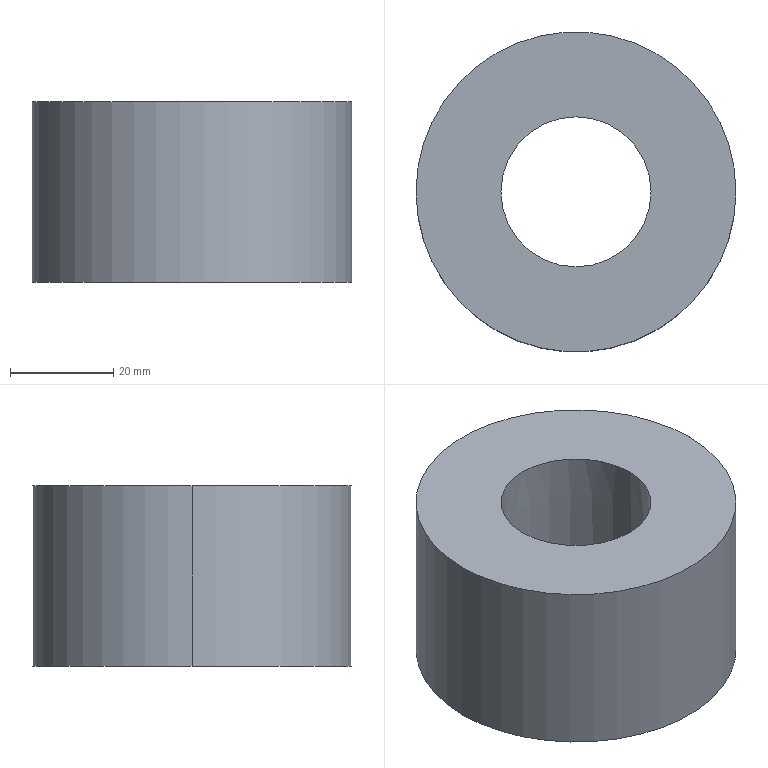Component | SolidWorks | JF21-80.1-1-3(_)-1-SOLID15-1 | 1 solid | 6 faces | box 62 x 62 x 35 mm | volume 80600 mm3 | cone 2 | cylinder 2 | plane 2 | commonest cylinder face diameters 62 x2
STEP:
#1=COLOUR_RGB('',0.7922,0.8196,0.9333);
#2=FILL_AREA_STYLE_COLOUR('',#1);
#3=FILL_AREA_STYLE('',(#2));
#4=SURFACE_STYLE_FILL_AREA(#3);
#5=SURFACE_SIDE_STYLE('',(#4));
#6=SURFACE_STYLE_USAGE(.BOTH.,#5);
#7=PRESENTATION_STYLE_ASSIGNMENT((#6));
#8=CARTESIAN_POINT('',(0.5728,-39.37,30.709));
#9=VERTEX_POINT('',#8);
#10=CARTESIAN_POINT('',(-0.5728,-39.37,30.709));
#11=VERTEX_POINT('',#10);
#12=CARTESIAN_POINT('',(0.,-39.37,30.709));
#13=DIRECTION('',(0.,0.,-1.));
#14=DIRECTION('',(-1.,0.,0.));
#15=AXIS2_PLACEMENT_3D('',#12,#13,#14);
#16=CIRCLE('',#15,0.5728);
#17=EDGE_CURVE('',#9,#11,#16,.T.);
#18=ORIENTED_EDGE('',*,*,#17,.F.);
#19=CARTESIAN_POINT('',(0.6158,-39.37,29.331));
#20=VERTEX_POINT('',#19);
#21=CARTESIAN_POINT('',(0.6158,-39.37,29.331));
#22=DIRECTION('',(-0.0312,-0.,0.9995));
#23=VECTOR('',#22,39.37);
#24=LINE('',#21,#23);
#25=EDGE_CURVE('',#20,#9,#24,.T.);
#26=ORIENTED_EDGE('',*,*,#25,.F.);
#27=CARTESIAN_POINT('',(-0.6158,-39.37,29.331));
#28=VERTEX_POINT('',#27);
#29=CARTESIAN_POINT('',(0.,-39.37,29.331));
#30=DIRECTION('',(0.,0.,-1.));
#31=DIRECTION('',(-1.,0.,0.));
#32=AXIS2_PLACEMENT_3D('',#29,#30,#31);
#33=CIRCLE('',#32,0.6158);
#34=EDGE_CURVE('',#20,#28,#33,.T.);
#35=ORIENTED_EDGE('',*,*,#34,.T.);
#36=CARTESIAN_POINT('',(-0.6158,-39.37,29.331));
#37=DIRECTION('',(0.0312,0.,0.9995));
#38=VECTOR('',#37,39.37);
#39=LINE('',#36,#38);
#40=EDGE_CURVE('',#28,#11,#39,.T.);
#41=ORIENTED_EDGE('',*,*,#40,.T.);
#42=EDGE_LOOP('',(#18,#26,#35,#41));
#43=FACE_OUTER_BOUND('',#42,.T.);
#44=CARTESIAN_POINT('',(0.,-39.37,29.331));
#45=DIRECTION('',(0.,0.,-1.));
#46=DIRECTION('',(1.,0.,0.));
#47=AXIS2_PLACEMENT_3D('',#44,#45,#46);
#48=CONICAL_SURFACE('',#47,0.6158,0.03121);
#49=ADVANCED_FACE('',(#43),#48,.F.);
#50=CARTESIAN_POINT('',(1.22,-39.37,30.709));
#51=VERTEX_POINT('',#50);
#52=CARTESIAN_POINT('',(-1.22,-39.37,30.709));
#53=VERTEX_POINT('',#52);
#54=CARTESIAN_POINT('',(0.,-39.37,30.709));
#55=DIRECTION('',(0.,0.,1.));
#56=DIRECTION('',(1.,0.,0.));
#57=AXIS2_PLACEMENT_3D('',#54,#55,#56);
#58=CIRCLE('',#57,1.22);
#59=EDGE_CURVE('',#51,#53,#58,.T.);
#60=ORIENTED_EDGE('',*,*,#59,.F.);
#61=CARTESIAN_POINT('',(1.22,-39.37,29.331));
#62=VERTEX_POINT('',#61);
#63=CARTESIAN_POINT('',(1.22,-39.37,30.709));
#64=DIRECTION('',(0.,0.,1.));
#65=VECTOR('',#64,39.37);
#66=LINE('',#63,#65);
#67=EDGE_CURVE('',#62,#51,#66,.T.);
#68=ORIENTED_EDGE('',*,*,#67,.F.);
#69=CARTESIAN_POINT('',(-1.22,-39.37,29.331));
#70=VERTEX_POINT('',#69);
#71=CARTESIAN_POINT('',(0.,-39.37,29.331));
#72=DIRECTION('',(0.,0.,1.));
#73=DIRECTION('',(1.,0.,0.));
#74=AXIS2_PLACEMENT_3D('',#71,#72,#73);
#75=CIRCLE('',#74,1.22);
#76=EDGE_CURVE('',#62,#70,#75,.T.);
#77=ORIENTED_EDGE('',*,*,#76,.T.);
#78=CARTESIAN_POINT('',(-1.22,-39.37,30.709));
#79=DIRECTION('',(0.,0.,1.));
#80=VECTOR('',#79,39.37);
#81=LINE('',#78,#80);
#82=EDGE_CURVE('',#70,#53,#81,.T.);
#83=ORIENTED_EDGE('',*,*,#82,.T.);
#84=EDGE_LOOP('',(#60,#68,#77,#83));
#85=FACE_OUTER_BOUND('',#84,.T.);
#86=CARTESIAN_POINT('',(0.,-39.37,30.709));
#87=DIRECTION('',(0.,0.,-1.));
#88=DIRECTION('',(1.,0.,0.));
#89=AXIS2_PLACEMENT_3D('',#86,#87,#88);
#90=CYLINDRICAL_SURFACE('',#89,1.22);
#91=ADVANCED_FACE('',(#85),#90,.T.);
#92=ORIENTED_EDGE('',*,*,#67,.T.);
#93=CARTESIAN_POINT('',(0.,-39.37,30.709));
#94=DIRECTION('',(0.,0.,1.));
#95=DIRECTION('',(1.,0.,0.));
#96=AXIS2_PLACEMENT_3D('',#93,#94,#95);
#97=CIRCLE('',#96,1.22);
#98=EDGE_CURVE('',#53,#51,#97,.T.);
#99=ORIENTED_EDGE('',*,*,#98,.F.);
#100=ORIENTED_EDGE('',*,*,#82,.F.);
#101=CARTESIAN_POINT('',(0.,-39.37,29.331));
#102=DIRECTION('',(0.,0.,1.));
#103=DIRECTION('',(1.,0.,0.));
#104=AXIS2_PLACEMENT_3D('',#101,#102,#103);
#105=CIRCLE('',#104,1.22);
#106=EDGE_CURVE('',#70,#62,#105,.T.);
#107=ORIENTED_EDGE('',*,*,#106,.T.);
#108=EDGE_LOOP('',(#92,#99,#100,#107));
#109=FACE_OUTER_BOUND('',#108,.T.);
#110=CARTESIAN_POINT('',(0.,-39.37,30.709));
#111=DIRECTION('',(0.,0.,-1.));
#112=DIRECTION('',(1.,0.,0.));
#113=AXIS2_PLACEMENT_3D('',#110,#111,#112);
#114=CYLINDRICAL_SURFACE('',#113,1.22);
#115=ADVANCED_FACE('',(#109),#114,.T.);
#116=CARTESIAN_POINT('',(0.,-39.37,30.709));
#117=DIRECTION('',(0.,0.,-1.));
#118=DIRECTION('',(-1.,0.,0.));
#119=AXIS2_PLACEMENT_3D('',#116,#117,#118);
#120=CIRCLE('',#119,0.5728);
#121=EDGE_CURVE('',#11,#9,#120,.T.);
#122=ORIENTED_EDGE('',*,*,#121,.T.);
#123=ORIENTED_EDGE('',*,*,#17,.T.);
#124=EDGE_LOOP('',(#122,#123));
#125=FACE_BOUND('',#124,.T.);
#126=ORIENTED_EDGE('',*,*,#98,.T.);
#127=ORIENTED_EDGE('',*,*,#59,.T.);
#128=EDGE_LOOP('',(#126,#127));
#129=FACE_OUTER_BOUND('',#128,.T.);
#130=CARTESIAN_POINT('',(0.,-39.37,30.709));
#131=DIRECTION('',(0.,0.,1.));
#132=DIRECTION('',(-1.,0.,0.));
#133=AXIS2_PLACEMENT_3D('',#130,#131,#132);
#134=PLANE('',#133);
#135=ADVANCED_FACE('',(#125,#129),#134,.T.);
#136=CARTESIAN_POINT('',(0.,-39.37,29.331));
#137=DIRECTION('',(0.,0.,-1.));
#138=DIRECTION('',(-1.,0.,0.));
#139=AXIS2_PLACEMENT_3D('',#136,#137,#138);
#140=CIRCLE('',#139,0.6158);
#141=EDGE_CURVE('',#28,#20,#140,.T.);
#142=ORIENTED_EDGE('',*,*,#141,.F.);
#143=ORIENTED_EDGE('',*,*,#34,.F.);
#144=EDGE_LOOP('',(#142,#143));
#145=FACE_BOUND('',#144,.T.);
#146=ORIENTED_EDGE('',*,*,#106,.F.);
#147=ORIENTED_EDGE('',*,*,#76,.F.);
#148=EDGE_LOOP('',(#146,#147));
#149=FACE_OUTER_BOUND('',#148,.T.);
#150=CARTESIAN_POINT('',(0.,-39.37,29.331));
#151=DIRECTION('',(0.,0.,1.));
#152=DIRECTION('',(-1.,0.,0.));
#153=AXIS2_PLACEMENT_3D('',#150,#151,#152);
#154=PLANE('',#153);
#155=ADVANCED_FACE('',(#145,#149),#154,.F.);
#156=ORIENTED_EDGE('',*,*,#25,.T.);
#157=ORIENTED_EDGE('',*,*,#121,.F.);
#158=ORIENTED_EDGE('',*,*,#40,.F.);
#159=ORIENTED_EDGE('',*,*,#141,.T.);
#160=EDGE_LOOP('',(#156,#157,#158,#159));
#161=FACE_OUTER_BOUND('',#160,.T.);
#162=CARTESIAN_POINT('',(0.,-39.37,29.331));
#163=DIRECTION('',(0.,0.,-1.));
#164=DIRECTION('',(1.,0.,0.));
#165=AXIS2_PLACEMENT_3D('',#162,#163,#164);
#166=CONICAL_SURFACE('',#165,0.6158,0.03121);
#167=ADVANCED_FACE('',(#161),#166,.F.);
#168=CLOSED_SHELL('',(#49,#91,#115,#135,#155,#167));
#169=MANIFOLD_SOLID_BREP('',#168);
#170=STYLED_ITEM('',(#7),#169);
#171=(LENGTH_UNIT()NAMED_UNIT(*)SI_UNIT($,.METRE.));
#172=LENGTH_MEASURE_WITH_UNIT(LENGTH_MEASURE(0.0254),#171);
#173=DIMENSIONAL_EXPONENTS(1.,0.,0.,0.,0.,0.,0.);
#174=(CONVERSION_BASED_UNIT('',#172)LENGTH_UNIT()NAMED_UNIT(#173));
#175=UNCERTAINTY_MEASURE_WITH_UNIT(LENGTH_MEASURE(0.00001),#174,'','');
#176=(NAMED_UNIT(*)PLANE_ANGLE_UNIT()SI_UNIT($,.RADIAN.));
#177=(NAMED_UNIT(*)SI_UNIT($,.STERADIAN.)SOLID_ANGLE_UNIT());
#178=(GEOMETRIC_REPRESENTATION_CONTEXT(3)GLOBAL_UNCERTAINTY_ASSIGNED_CONTEXT((#175))GLOBAL_UNIT_ASSIGNED_CONTEXT((#174,#176,#177))REPRESENTATION_CONTEXT('',''));
#179=MECHANICAL_DESIGN_GEOMETRIC_PRESENTATION_REPRESENTATION('',(#170),#178);
#180=PRESENTATION_LAYER_ASSIGNMENT('','',(#170));
#181=CARTESIAN_POINT('',(0.,0.,0.));
#182=DIRECTION('',(0.,0.,1.));
#183=DIRECTION('',(1.,0.,0.));
#184=AXIS2_PLACEMENT_3D('',#181,#182,#183);
#185=(LENGTH_UNIT()NAMED_UNIT(*)SI_UNIT($,.METRE.));
#186=LENGTH_MEASURE_WITH_UNIT(LENGTH_MEASURE(0.0254),#185);
#187=DIMENSIONAL_EXPONENTS(1.,0.,0.,0.,0.,0.,0.);
#188=(CONVERSION_BASED_UNIT('',#186)LENGTH_UNIT()NAMED_UNIT(#187));
#189=UNCERTAINTY_MEASURE_WITH_UNIT(LENGTH_MEASURE(0.00001),#188,'','');
#190=(NAMED_UNIT(*)PLANE_ANGLE_UNIT()SI_UNIT($,.RADIAN.));
#191=(NAMED_UNIT(*)SI_UNIT($,.STERADIAN.)SOLID_ANGLE_UNIT());
#192=(GEOMETRIC_REPRESENTATION_CONTEXT(3)GLOBAL_UNCERTAINTY_ASSIGNED_CONTEXT((#189))GLOBAL_UNIT_ASSIGNED_CONTEXT((#188,#190,#191))REPRESENTATION_CONTEXT('',''));
#193=ADVANCED_BREP_SHAPE_REPRESENTATION('',(#169,#184),#192);